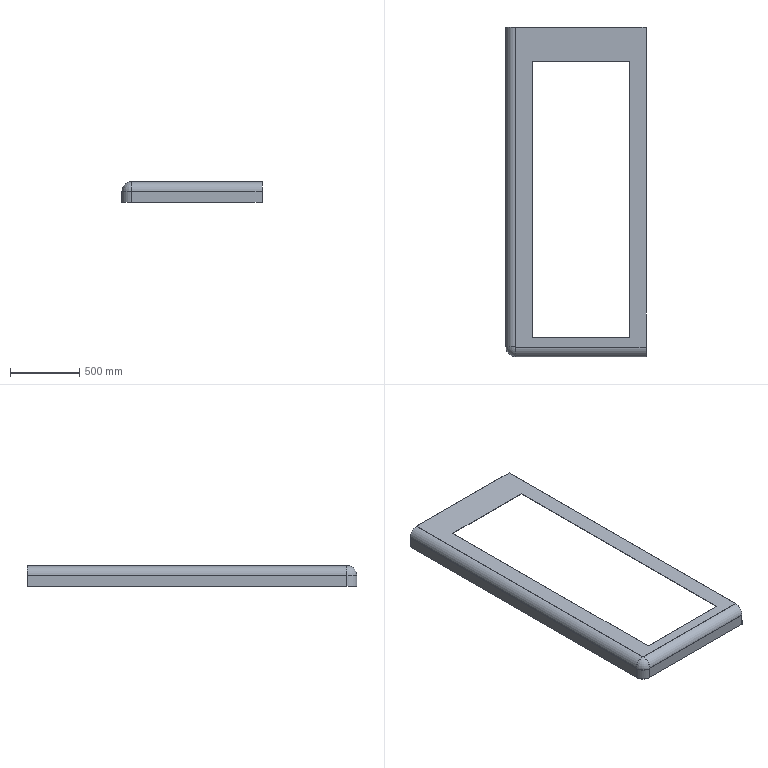Component | SolidWorks | A-SideAluminumCasingAssembly-1_A-SideAluminumCasing1-1 | 1 solid | 25 faces | box 1009.5 x 2375.5 x 149.5 mm | volume 4190304 mm3 | plane 17 | cylinder 6 | torus 2 | commonest cylinder face diameters 139 x2 133 x2 141 x1 135 x1
STEP:
#1=CARTESIAN_POINT('',(-0.2362,90.787,73.937));
#2=VERTEX_POINT('',#1);
#3=CARTESIAN_POINT('',(-0.2362,90.787,73.819));
#4=VERTEX_POINT('',#3);
#5=CARTESIAN_POINT('',(-0.2362,90.787,73.819));
#6=DIRECTION('',(0.,-0.,-1.));
#7=VECTOR('',#6,39.37);
#8=LINE('',#5,#7);
#9=EDGE_CURVE('',#2,#4,#8,.T.);
#10=ORIENTED_EDGE('',*,*,#9,.F.);
#11=CARTESIAN_POINT('',(-0.2362,0.,73.937));
#12=VERTEX_POINT('',#11);
#13=CARTESIAN_POINT('',(-0.2362,0.,73.937));
#14=DIRECTION('',(0.,-1.,0.));
#15=VECTOR('',#14,39.37);
#16=LINE('',#13,#15);
#17=EDGE_CURVE('',#2,#12,#16,.T.);
#18=ORIENTED_EDGE('',*,*,#17,.T.);
#19=CARTESIAN_POINT('',(-0.2362,0.,73.819));
#20=VERTEX_POINT('',#19);
#21=CARTESIAN_POINT('',(-0.2362,0.,73.819));
#22=DIRECTION('',(0.,-0.,-1.));
#23=VECTOR('',#22,39.37);
#24=LINE('',#21,#23);
#25=EDGE_CURVE('',#12,#20,#24,.T.);
#26=ORIENTED_EDGE('',*,*,#25,.T.);
#27=CARTESIAN_POINT('',(-0.2362,0.,73.819));
#28=DIRECTION('',(0.,-1.,0.));
#29=VECTOR('',#28,39.37);
#30=LINE('',#27,#29);
#31=EDGE_CURVE('',#4,#20,#30,.T.);
#32=ORIENTED_EDGE('',*,*,#31,.F.);
#33=EDGE_LOOP('',(#10,#18,#26,#32));
#34=FACE_OUTER_BOUND('',#33,.T.);
#35=CARTESIAN_POINT('',(-0.2362,0.,73.819));
#36=DIRECTION('',(1.,0.,0.));
#37=DIRECTION('',(0.,-1.,0.));
#38=AXIS2_PLACEMENT_3D('',#35,#36,#37);
#39=PLANE('',#38);
#40=ADVANCED_FACE('',(#34),#39,.T.);
#41=CARTESIAN_POINT('',(-37.244,90.787,73.937));
#42=VERTEX_POINT('',#41);
#43=CARTESIAN_POINT('',(-37.244,90.787,73.937));
#44=DIRECTION('',(1.,0.,0.));
#45=VECTOR('',#44,39.37);
#46=LINE('',#43,#45);
#47=EDGE_CURVE('',#42,#2,#46,.T.);
#48=ORIENTED_EDGE('',*,*,#47,.T.);
#49=ORIENTED_EDGE('',*,*,#9,.T.);
#50=CARTESIAN_POINT('',(-37.244,90.787,73.819));
#51=VERTEX_POINT('',#50);
#52=CARTESIAN_POINT('',(-37.244,90.787,73.819));
#53=DIRECTION('',(1.,0.,0.));
#54=VECTOR('',#53,39.37);
#55=LINE('',#52,#54);
#56=EDGE_CURVE('',#51,#4,#55,.T.);
#57=ORIENTED_EDGE('',*,*,#56,.F.);
#58=CARTESIAN_POINT('',(-37.244,90.787,73.819));
#59=DIRECTION('',(0.,-0.,-1.));
#60=VECTOR('',#59,39.37);
#61=LINE('',#58,#60);
#62=EDGE_CURVE('',#42,#51,#61,.T.);
#63=ORIENTED_EDGE('',*,*,#62,.F.);
#64=EDGE_LOOP('',(#48,#49,#57,#63));
#65=FACE_OUTER_BOUND('',#64,.T.);
#66=CARTESIAN_POINT('',(-37.244,90.787,73.819));
#67=DIRECTION('',(-0.,1.,-0.));
#68=DIRECTION('',(1.,0.,0.));
#69=AXIS2_PLACEMENT_3D('',#66,#67,#68);
#70=PLANE('',#69);
#71=ADVANCED_FACE('',(#65),#70,.T.);
#72=CARTESIAN_POINT('',(-32.48,2.736,73.819));
#73=VERTEX_POINT('',#72);
#74=CARTESIAN_POINT('',(-32.48,81.083,73.819));
#75=VERTEX_POINT('',#74);
#76=CARTESIAN_POINT('',(-32.48,0.,73.819));
#77=DIRECTION('',(-0.,1.,-0.));
#78=VECTOR('',#77,39.37);
#79=LINE('',#76,#78);
#80=EDGE_CURVE('',#73,#75,#79,.T.);
#81=ORIENTED_EDGE('',*,*,#80,.F.);
#82=CARTESIAN_POINT('',(-4.921,2.736,73.819));
#83=VERTEX_POINT('',#82);
#84=CARTESIAN_POINT('',(-37.244,2.736,73.819));
#85=DIRECTION('',(-1.,-0.,-0.));
#86=VECTOR('',#85,39.37);
#87=LINE('',#84,#86);
#88=EDGE_CURVE('',#83,#73,#87,.T.);
#89=ORIENTED_EDGE('',*,*,#88,.F.);
#90=CARTESIAN_POINT('',(-4.921,81.083,73.819));
#91=VERTEX_POINT('',#90);
#92=CARTESIAN_POINT('',(-4.921,0.,73.819));
#93=DIRECTION('',(0.,-1.,0.));
#94=VECTOR('',#93,39.37);
#95=LINE('',#92,#94);
#96=EDGE_CURVE('',#91,#83,#95,.T.);
#97=ORIENTED_EDGE('',*,*,#96,.F.);
#98=CARTESIAN_POINT('',(-37.244,81.083,73.819));
#99=DIRECTION('',(1.,0.,0.));
#100=VECTOR('',#99,39.37);
#101=LINE('',#98,#100);
#102=EDGE_CURVE('',#75,#91,#101,.T.);
#103=ORIENTED_EDGE('',*,*,#102,.F.);
#104=EDGE_LOOP('',(#81,#89,#97,#103));
#105=FACE_BOUND('',#104,.T.);
#106=CARTESIAN_POINT('',(-37.205,0.,73.819));
#107=VERTEX_POINT('',#106);
#108=CARTESIAN_POINT('',(-37.244,0.,73.819));
#109=DIRECTION('',(-1.,-0.,-0.));
#110=VECTOR('',#109,39.37);
#111=LINE('',#108,#110);
#112=EDGE_CURVE('',#20,#107,#111,.T.);
#113=ORIENTED_EDGE('',*,*,#112,.T.);
#114=CARTESIAN_POINT('',(-37.244,0.03937,73.819));
#115=VERTEX_POINT('',#114);
#116=CARTESIAN_POINT('',(-37.205,0.03937,73.819));
#117=DIRECTION('',(0.,-0.,-1.));
#118=DIRECTION('',(-1.,-0.,0.));
#119=AXIS2_PLACEMENT_3D('',#116,#117,#118);
#120=CIRCLE('',#119,0.03937);
#121=EDGE_CURVE('',#107,#115,#120,.T.);
#122=ORIENTED_EDGE('',*,*,#121,.T.);
#123=CARTESIAN_POINT('',(-37.244,0.,73.819));
#124=DIRECTION('',(-0.,1.,-0.));
#125=VECTOR('',#124,39.37);
#126=LINE('',#123,#125);
#127=EDGE_CURVE('',#115,#51,#126,.T.);
#128=ORIENTED_EDGE('',*,*,#127,.T.);
#129=ORIENTED_EDGE('',*,*,#56,.T.);
#130=ORIENTED_EDGE('',*,*,#31,.T.);
#131=EDGE_LOOP('',(#113,#122,#128,#129,#130));
#132=FACE_OUTER_BOUND('',#131,.T.);
#133=CARTESIAN_POINT('',(-37.244,0.,73.819));
#134=DIRECTION('',(0.,-0.,-1.));
#135=DIRECTION('',(-1.,-0.,-0.));
#136=AXIS2_PLACEMENT_3D('',#133,#134,#135);
#137=PLANE('',#136);
#138=ADVANCED_FACE('',(#105,#132),#137,.T.);
#139=CARTESIAN_POINT('',(-32.48,2.736,73.937));
#140=VERTEX_POINT('',#139);
#141=CARTESIAN_POINT('',(-4.921,2.736,73.937));
#142=VERTEX_POINT('',#141);
#143=CARTESIAN_POINT('',(-32.48,2.736,73.937));
#144=DIRECTION('',(1.,0.,0.));
#145=VECTOR('',#144,39.37);
#146=LINE('',#143,#145);
#147=EDGE_CURVE('',#140,#142,#146,.T.);
#148=ORIENTED_EDGE('',*,*,#147,.F.);
#149=CARTESIAN_POINT('',(-32.48,81.083,73.937));
#150=VERTEX_POINT('',#149);
#151=CARTESIAN_POINT('',(-32.48,2.736,73.937));
#152=DIRECTION('',(0.,-1.,0.));
#153=VECTOR('',#152,39.37);
#154=LINE('',#151,#153);
#155=EDGE_CURVE('',#150,#140,#154,.T.);
#156=ORIENTED_EDGE('',*,*,#155,.F.);
#157=CARTESIAN_POINT('',(-4.921,81.083,73.937));
#158=VERTEX_POINT('',#157);
#159=CARTESIAN_POINT('',(-32.48,81.083,73.937));
#160=DIRECTION('',(-1.,-0.,-0.));
#161=VECTOR('',#160,39.37);
#162=LINE('',#159,#161);
#163=EDGE_CURVE('',#158,#150,#162,.T.);
#164=ORIENTED_EDGE('',*,*,#163,.F.);
#165=CARTESIAN_POINT('',(-4.921,2.736,73.937));
#166=DIRECTION('',(-0.,1.,-0.));
#167=VECTOR('',#166,39.37);
#168=LINE('',#165,#167);
#169=EDGE_CURVE('',#142,#158,#168,.T.);
#170=ORIENTED_EDGE('',*,*,#169,.F.);
#171=EDGE_LOOP('',(#148,#156,#164,#170));
#172=FACE_BOUND('',#171,.T.);
#173=CARTESIAN_POINT('',(-37.244,0.03937,73.937));
#174=VERTEX_POINT('',#173);
#175=CARTESIAN_POINT('',(-37.244,0.,73.937));
#176=DIRECTION('',(-0.,1.,-0.));
#177=VECTOR('',#176,39.37);
#178=LINE('',#175,#177);
#179=EDGE_CURVE('',#174,#42,#178,.T.);
#180=ORIENTED_EDGE('',*,*,#179,.F.);
#181=CARTESIAN_POINT('',(-37.205,0.,73.937));
#182=VERTEX_POINT('',#181);
#183=CARTESIAN_POINT('',(-37.205,0.03937,73.937));
#184=DIRECTION('',(-0.,0.,1.));
#185=DIRECTION('',(-1.,-0.,0.));
#186=AXIS2_PLACEMENT_3D('',#183,#184,#185);
#187=CIRCLE('',#186,0.03937);
#188=EDGE_CURVE('',#174,#182,#187,.T.);
#189=ORIENTED_EDGE('',*,*,#188,.T.);
#190=CARTESIAN_POINT('',(-37.244,0.,73.937));
#191=DIRECTION('',(-1.,-0.,-0.));
#192=VECTOR('',#191,39.37);
#193=LINE('',#190,#192);
#194=EDGE_CURVE('',#12,#182,#193,.T.);
#195=ORIENTED_EDGE('',*,*,#194,.F.);
#196=ORIENTED_EDGE('',*,*,#17,.F.);
#197=ORIENTED_EDGE('',*,*,#47,.F.);
#198=EDGE_LOOP('',(#180,#189,#195,#196,#197));
#199=FACE_OUTER_BOUND('',#198,.T.);
#200=CARTESIAN_POINT('',(-37.244,0.,73.937));
#201=DIRECTION('',(0.,-0.,-1.));
#202=DIRECTION('',(-1.,-0.,-0.));
#203=AXIS2_PLACEMENT_3D('',#200,#201,#202);
#204=PLANE('',#203);
#205=ADVANCED_FACE('',(#172,#199),#204,.F.);
#206=CARTESIAN_POINT('',(-0.2362,-2.618,71.201));
#207=VERTEX_POINT('',#206);
#208=CARTESIAN_POINT('',(-0.2362,-2.736,71.201));
#209=VERTEX_POINT('',#208);
#210=CARTESIAN_POINT('',(-0.2362,-2.736,71.201));
#211=DIRECTION('',(0.,-1.,0.));
#212=VECTOR('',#211,39.37);
#213=LINE('',#210,#212);
#214=EDGE_CURVE('',#207,#209,#213,.T.);
#215=ORIENTED_EDGE('',*,*,#214,.F.);
#216=CARTESIAN_POINT('',(-0.2362,0.,71.201));
#217=DIRECTION('',(1.,0.,0.));
#218=DIRECTION('',(-0.,0.,1.));
#219=AXIS2_PLACEMENT_3D('',#216,#217,#218);
#220=CIRCLE('',#219,2.618);
#221=EDGE_CURVE('',#20,#207,#220,.T.);
#222=ORIENTED_EDGE('',*,*,#221,.F.);
#223=ORIENTED_EDGE('',*,*,#25,.F.);
#224=CARTESIAN_POINT('',(-0.2362,0.,71.201));
#225=DIRECTION('',(1.,0.,0.));
#226=DIRECTION('',(-0.,0.,1.));
#227=AXIS2_PLACEMENT_3D('',#224,#225,#226);
#228=CIRCLE('',#227,2.736);
#229=EDGE_CURVE('',#12,#209,#228,.T.);
#230=ORIENTED_EDGE('',*,*,#229,.T.);
#231=EDGE_LOOP('',(#215,#222,#223,#230));
#232=FACE_OUTER_BOUND('',#231,.T.);
#233=CARTESIAN_POINT('',(-0.2362,0.,71.201));
#234=DIRECTION('',(1.,0.,0.));
#235=DIRECTION('',(0.,-0.,-1.));
#236=AXIS2_PLACEMENT_3D('',#233,#234,#235);
#237=PLANE('',#236);
#238=ADVANCED_FACE('',(#232),#237,.T.);
#239=ORIENTED_EDGE('',*,*,#194,.T.);
#240=CARTESIAN_POINT('',(-37.205,-2.736,71.201));
#241=VERTEX_POINT('',#240);
#242=CARTESIAN_POINT('',(-37.205,0.,71.201));
#243=DIRECTION('',(-1.,-0.,-0.));
#244=DIRECTION('',(0.,0.,1.));
#245=AXIS2_PLACEMENT_3D('',#242,#243,#244);
#246=CIRCLE('',#245,2.736);
#247=EDGE_CURVE('',#241,#182,#246,.T.);
#248=ORIENTED_EDGE('',*,*,#247,.F.);
#249=CARTESIAN_POINT('',(-0.2362,-2.736,71.201));
#250=DIRECTION('',(1.,0.,0.));
#251=VECTOR('',#250,39.37);
#252=LINE('',#249,#251);
#253=EDGE_CURVE('',#241,#209,#252,.T.);
#254=ORIENTED_EDGE('',*,*,#253,.T.);
#255=ORIENTED_EDGE('',*,*,#229,.F.);
#256=EDGE_LOOP('',(#239,#248,#254,#255));
#257=FACE_OUTER_BOUND('',#256,.T.);
#258=CARTESIAN_POINT('',(-37.205,0.,71.201));
#259=DIRECTION('',(-1.,-0.,-0.));
#260=DIRECTION('',(0.,-1.,0.));
#261=AXIS2_PLACEMENT_3D('',#258,#259,#260);
#262=CYLINDRICAL_SURFACE('',#261,2.736);
#263=ADVANCED_FACE('',(#257),#262,.T.);
#264=ORIENTED_EDGE('',*,*,#112,.F.);
#265=ORIENTED_EDGE('',*,*,#221,.T.);
#266=CARTESIAN_POINT('',(-37.205,-2.618,71.201));
#267=VERTEX_POINT('',#266);
#268=CARTESIAN_POINT('',(-0.2362,-2.618,71.201));
#269=DIRECTION('',(-1.,-0.,-0.));
#270=VECTOR('',#269,39.37);
#271=LINE('',#268,#270);
#272=EDGE_CURVE('',#207,#267,#271,.T.);
#273=ORIENTED_EDGE('',*,*,#272,.T.);
#274=CARTESIAN_POINT('',(-37.205,0.,71.201));
#275=DIRECTION('',(-1.,-0.,-0.));
#276=DIRECTION('',(0.,0.,1.));
#277=AXIS2_PLACEMENT_3D('',#274,#275,#276);
#278=CIRCLE('',#277,2.618);
#279=EDGE_CURVE('',#267,#107,#278,.T.);
#280=ORIENTED_EDGE('',*,*,#279,.T.);
#281=EDGE_LOOP('',(#264,#265,#273,#280));
#282=FACE_OUTER_BOUND('',#281,.T.);
#283=CARTESIAN_POINT('',(-37.205,0.,71.201));
#284=DIRECTION('',(-1.,-0.,-0.));
#285=DIRECTION('',(0.,-1.,0.));
#286=AXIS2_PLACEMENT_3D('',#283,#284,#285);
#287=CYLINDRICAL_SURFACE('',#286,2.618);
#288=ADVANCED_FACE('',(#282),#287,.F.);
#289=ORIENTED_EDGE('',*,*,#214,.T.);
#290=CARTESIAN_POINT('',(-0.2362,-2.736,68.051));
#291=VERTEX_POINT('',#290);
#292=CARTESIAN_POINT('',(-0.2362,-2.736,73.819));
#293=DIRECTION('',(-0.,0.,1.));
#294=VECTOR('',#293,39.37);
#295=LINE('',#292,#294);
#296=EDGE_CURVE('',#291,#209,#295,.T.);
#297=ORIENTED_EDGE('',*,*,#296,.F.);
#298=CARTESIAN_POINT('',(-0.2362,-2.618,68.051));
#299=VERTEX_POINT('',#298);
#300=CARTESIAN_POINT('',(-0.2362,-2.736,68.051));
#301=DIRECTION('',(-0.,1.,-0.));
#302=VECTOR('',#301,39.37);
#303=LINE('',#300,#302);
#304=EDGE_CURVE('',#291,#299,#303,.T.);
#305=ORIENTED_EDGE('',*,*,#304,.T.);
#306=CARTESIAN_POINT('',(-0.2362,-2.618,73.819));
#307=DIRECTION('',(-0.,0.,1.));
#308=VECTOR('',#307,39.37);
#309=LINE('',#306,#308);
#310=EDGE_CURVE('',#299,#207,#309,.T.);
#311=ORIENTED_EDGE('',*,*,#310,.T.);
#312=EDGE_LOOP('',(#289,#297,#305,#311));
#313=FACE_OUTER_BOUND('',#312,.T.);
#314=CARTESIAN_POINT('',(-0.2362,-2.736,73.819));
#315=DIRECTION('',(-1.,-0.,-0.));
#316=DIRECTION('',(-0.,0.,1.));
#317=AXIS2_PLACEMENT_3D('',#314,#315,#316);
#318=PLANE('',#317);
#319=ADVANCED_FACE('',(#313),#318,.F.);
#320=ORIENTED_EDGE('',*,*,#253,.F.);
#321=CARTESIAN_POINT('',(-37.205,-2.736,68.051));
#322=VERTEX_POINT('',#321);
#323=CARTESIAN_POINT('',(-37.205,-2.736,73.819));
#324=DIRECTION('',(0.,-0.,-1.));
#325=VECTOR('',#324,39.37);
#326=LINE('',#323,#325);
#327=EDGE_CURVE('',#241,#322,#326,.T.);
#328=ORIENTED_EDGE('',*,*,#327,.T.);
#329=CARTESIAN_POINT('',(-37.244,-2.736,68.051));
#330=DIRECTION('',(1.,0.,0.));
#331=VECTOR('',#330,39.37);
#332=LINE('',#329,#331);
#333=EDGE_CURVE('',#322,#291,#332,.T.);
#334=ORIENTED_EDGE('',*,*,#333,.T.);
#335=ORIENTED_EDGE('',*,*,#296,.T.);
#336=EDGE_LOOP('',(#320,#328,#334,#335));
#337=FACE_OUTER_BOUND('',#336,.T.);
#338=CARTESIAN_POINT('',(-37.244,-2.736,73.819));
#339=DIRECTION('',(-0.,1.,-0.));
#340=DIRECTION('',(0.,-0.,-1.));
#341=AXIS2_PLACEMENT_3D('',#338,#339,#340);
#342=PLANE('',#341);
#343=ADVANCED_FACE('',(#337),#342,.F.);
#344=CARTESIAN_POINT('',(-37.205,-2.618,68.051));
#345=VERTEX_POINT('',#344);
#346=CARTESIAN_POINT('',(-37.205,-2.618,68.051));
#347=DIRECTION('',(0.,-0.,-1.));
#348=VECTOR('',#347,39.37);
#349=LINE('',#346,#348);
#350=EDGE_CURVE('',#267,#345,#349,.T.);
#351=ORIENTED_EDGE('',*,*,#350,.F.);
#352=ORIENTED_EDGE('',*,*,#272,.F.);
#353=ORIENTED_EDGE('',*,*,#310,.F.);
#354=CARTESIAN_POINT('',(-0.2362,-2.618,68.051));
#355=DIRECTION('',(1.,0.,0.));
#356=VECTOR('',#355,39.37);
#357=LINE('',#354,#356);
#358=EDGE_CURVE('',#345,#299,#357,.T.);
#359=ORIENTED_EDGE('',*,*,#358,.F.);
#360=EDGE_LOOP('',(#351,#352,#353,#359));
#361=FACE_OUTER_BOUND('',#360,.T.);
#362=CARTESIAN_POINT('',(-37.244,-2.618,73.819));
#363=DIRECTION('',(-0.,1.,-0.));
#364=DIRECTION('',(0.,-0.,-1.));
#365=AXIS2_PLACEMENT_3D('',#362,#363,#364);
#366=PLANE('',#365);
#367=ADVANCED_FACE('',(#361),#366,.T.);
#368=ORIENTED_EDGE('',*,*,#358,.T.);
#369=ORIENTED_EDGE('',*,*,#304,.F.);
#370=ORIENTED_EDGE('',*,*,#333,.F.);
#371=CARTESIAN_POINT('',(-39.98,0.03937,68.051));
#372=VERTEX_POINT('',#371);
#373=CARTESIAN_POINT('',(-37.205,0.03937,68.051));
#374=DIRECTION('',(0.,-0.,-1.));
#375=DIRECTION('',(0.,-1.,0.));
#376=AXIS2_PLACEMENT_3D('',#373,#374,#375);
#377=CIRCLE('',#376,2.776);
#378=EDGE_CURVE('',#322,#372,#377,.T.);
#379=ORIENTED_EDGE('',*,*,#378,.T.);
#380=CARTESIAN_POINT('',(-39.98,90.787,68.051));
#381=VERTEX_POINT('',#380);
#382=CARTESIAN_POINT('',(-39.98,0.,68.051));
#383=DIRECTION('',(0.,-1.,0.));
#384=VECTOR('',#383,39.37);
#385=LINE('',#382,#384);
#386=EDGE_CURVE('',#381,#372,#385,.T.);
#387=ORIENTED_EDGE('',*,*,#386,.F.);
#388=CARTESIAN_POINT('',(-39.862,90.787,68.051));
#389=VERTEX_POINT('',#388);
#390=CARTESIAN_POINT('',(-39.98,90.787,68.051));
#391=DIRECTION('',(1.,0.,-0.));
#392=VECTOR('',#391,39.37);
#393=LINE('',#390,#392);
#394=EDGE_CURVE('',#381,#389,#393,.T.);
#395=ORIENTED_EDGE('',*,*,#394,.T.);
#396=CARTESIAN_POINT('',(-39.862,0.03937,68.051));
#397=VERTEX_POINT('',#396);
#398=CARTESIAN_POINT('',(-39.862,0.03937,68.051));
#399=DIRECTION('',(0.,-1.,0.));
#400=VECTOR('',#399,39.37);
#401=LINE('',#398,#400);
#402=EDGE_CURVE('',#389,#397,#401,.T.);
#403=ORIENTED_EDGE('',*,*,#402,.T.);
#404=CARTESIAN_POINT('',(-37.205,0.03937,68.051));
#405=DIRECTION('',(0.,-0.,-1.));
#406=DIRECTION('',(0.,-1.,0.));
#407=AXIS2_PLACEMENT_3D('',#404,#405,#406);
#408=CIRCLE('',#407,2.657);
#409=EDGE_CURVE('',#345,#397,#408,.T.);
#410=ORIENTED_EDGE('',*,*,#409,.F.);
#411=EDGE_LOOP('',(#368,#369,#370,#379,#387,#395,#403,#410));
#412=FACE_OUTER_BOUND('',#411,.T.);
#413=CARTESIAN_POINT('',(-0.2362,-2.736,68.051));
#414=DIRECTION('',(-0.,0.,1.));
#415=DIRECTION('',(-0.,1.,-0.));
#416=AXIS2_PLACEMENT_3D('',#413,#414,#415);
#417=PLANE('',#416);
#418=ADVANCED_FACE('',(#412),#417,.F.);
#419=CARTESIAN_POINT('',(-39.862,90.787,71.201));
#420=VERTEX_POINT('',#419);
#421=CARTESIAN_POINT('',(-37.244,90.787,71.201));
#422=DIRECTION('',(-0.,1.,-0.));
#423=DIRECTION('',(0.,-0.,-1.));
#424=AXIS2_PLACEMENT_3D('',#421,#422,#423);
#425=CIRCLE('',#424,2.618);
#426=EDGE_CURVE('',#420,#51,#425,.T.);
#427=ORIENTED_EDGE('',*,*,#426,.F.);
#428=CARTESIAN_POINT('',(-39.98,90.787,71.201));
#429=VERTEX_POINT('',#428);
#430=CARTESIAN_POINT('',(-39.862,90.787,71.201));
#431=DIRECTION('',(-1.,-0.,0.));
#432=VECTOR('',#431,39.37);
#433=LINE('',#430,#432);
#434=EDGE_CURVE('',#420,#429,#433,.T.);
#435=ORIENTED_EDGE('',*,*,#434,.T.);
#436=CARTESIAN_POINT('',(-37.244,90.787,71.201));
#437=DIRECTION('',(-0.,1.,-0.));
#438=DIRECTION('',(0.,-0.,-1.));
#439=AXIS2_PLACEMENT_3D('',#436,#437,#438);
#440=CIRCLE('',#439,2.736);
#441=EDGE_CURVE('',#429,#42,#440,.T.);
#442=ORIENTED_EDGE('',*,*,#441,.T.);
#443=ORIENTED_EDGE('',*,*,#62,.T.);
#444=EDGE_LOOP('',(#427,#435,#442,#443));
#445=FACE_OUTER_BOUND('',#444,.T.);
#446=CARTESIAN_POINT('',(-37.244,90.787,71.201));
#447=DIRECTION('',(0.,-1.,0.));
#448=DIRECTION('',(-0.,0.,1.));
#449=AXIS2_PLACEMENT_3D('',#446,#447,#448);
#450=PLANE('',#449);
#451=ADVANCED_FACE('',(#445),#450,.F.);
#452=ORIENTED_EDGE('',*,*,#179,.T.);
#453=ORIENTED_EDGE('',*,*,#441,.F.);
#454=CARTESIAN_POINT('',(-39.98,0.03937,71.201));
#455=VERTEX_POINT('',#454);
#456=CARTESIAN_POINT('',(-39.98,0.03937,71.201));
#457=DIRECTION('',(0.,-1.,0.));
#458=VECTOR('',#457,39.37);
#459=LINE('',#456,#458);
#460=EDGE_CURVE('',#429,#455,#459,.T.);
#461=ORIENTED_EDGE('',*,*,#460,.T.);
#462=CARTESIAN_POINT('',(-37.244,0.03937,71.201));
#463=DIRECTION('',(0.,-1.,0.));
#464=DIRECTION('',(0.,-0.,-1.));
#465=AXIS2_PLACEMENT_3D('',#462,#463,#464);
#466=CIRCLE('',#465,2.736);
#467=EDGE_CURVE('',#174,#455,#466,.T.);
#468=ORIENTED_EDGE('',*,*,#467,.F.);
#469=EDGE_LOOP('',(#452,#453,#461,#468));
#470=FACE_OUTER_BOUND('',#469,.T.);
#471=CARTESIAN_POINT('',(-37.244,90.787,71.201));
#472=DIRECTION('',(-0.,1.,-0.));
#473=DIRECTION('',(-1.,-0.,0.));
#474=AXIS2_PLACEMENT_3D('',#471,#472,#473);
#475=CYLINDRICAL_SURFACE('',#474,2.736);
#476=ADVANCED_FACE('',(#470),#475,.T.);
#477=ORIENTED_EDGE('',*,*,#127,.F.);
#478=CARTESIAN_POINT('',(-39.862,0.03937,71.201));
#479=VERTEX_POINT('',#478);
#480=CARTESIAN_POINT('',(-37.244,0.03937,71.201));
#481=DIRECTION('',(0.,-1.,0.));
#482=DIRECTION('',(0.,-0.,-1.));
#483=AXIS2_PLACEMENT_3D('',#480,#481,#482);
#484=CIRCLE('',#483,2.618);
#485=EDGE_CURVE('',#115,#479,#484,.T.);
#486=ORIENTED_EDGE('',*,*,#485,.T.);
#487=CARTESIAN_POINT('',(-39.862,0.03937,71.201));
#488=DIRECTION('',(-0.,1.,-0.));
#489=VECTOR('',#488,39.37);
#490=LINE('',#487,#489);
#491=EDGE_CURVE('',#479,#420,#490,.T.);
#492=ORIENTED_EDGE('',*,*,#491,.T.);
#493=ORIENTED_EDGE('',*,*,#426,.T.);
#494=EDGE_LOOP('',(#477,#486,#492,#493));
#495=FACE_OUTER_BOUND('',#494,.T.);
#496=CARTESIAN_POINT('',(-37.244,90.787,71.201));
#497=DIRECTION('',(-0.,1.,-0.));
#498=DIRECTION('',(-1.,-0.,0.));
#499=AXIS2_PLACEMENT_3D('',#496,#497,#498);
#500=CYLINDRICAL_SURFACE('',#499,2.618);
#501=ADVANCED_FACE('',(#495),#500,.F.);
#502=ORIENTED_EDGE('',*,*,#434,.F.);
#503=CARTESIAN_POINT('',(-39.862,90.787,68.051));
#504=DIRECTION('',(-0.,-0.,-1.));
#505=VECTOR('',#504,39.37);
#506=LINE('',#503,#505);
#507=EDGE_CURVE('',#420,#389,#506,.T.);
#508=ORIENTED_EDGE('',*,*,#507,.T.);
#509=ORIENTED_EDGE('',*,*,#394,.F.);
#510=CARTESIAN_POINT('',(-39.98,90.787,73.819));
#511=DIRECTION('',(-0.,-0.,-1.));
#512=VECTOR('',#511,39.37);
#513=LINE('',#510,#512);
#514=EDGE_CURVE('',#429,#381,#513,.T.);
#515=ORIENTED_EDGE('',*,*,#514,.F.);
#516=EDGE_LOOP('',(#502,#508,#509,#515));
#517=FACE_OUTER_BOUND('',#516,.T.);
#518=CARTESIAN_POINT('',(-39.98,90.787,68.051));
#519=DIRECTION('',(0.,-1.,0.));
#520=DIRECTION('',(-1.,-0.,-0.));
#521=AXIS2_PLACEMENT_3D('',#518,#519,#520);
#522=PLANE('',#521);
#523=ADVANCED_FACE('',(#517),#522,.F.);
#524=ORIENTED_EDGE('',*,*,#460,.F.);
#525=ORIENTED_EDGE('',*,*,#514,.T.);
#526=ORIENTED_EDGE('',*,*,#386,.T.);
#527=CARTESIAN_POINT('',(-39.98,0.03937,73.819));
#528=DIRECTION('',(0.,0.,1.));
#529=VECTOR('',#528,39.37);
#530=LINE('',#527,#529);
#531=EDGE_CURVE('',#372,#455,#530,.T.);
#532=ORIENTED_EDGE('',*,*,#531,.T.);
#533=EDGE_LOOP('',(#524,#525,#526,#532));
#534=FACE_OUTER_BOUND('',#533,.T.);
#535=CARTESIAN_POINT('',(-39.98,0.,73.819));
#536=DIRECTION('',(1.,0.,-0.));
#537=DIRECTION('',(-0.,-0.,-1.));
#538=AXIS2_PLACEMENT_3D('',#535,#536,#537);
#539=PLANE('',#538);
#540=ADVANCED_FACE('',(#534),#539,.F.);
#541=ORIENTED_EDGE('',*,*,#507,.F.);
#542=ORIENTED_EDGE('',*,*,#491,.F.);
#543=CARTESIAN_POINT('',(-39.862,0.03937,73.819));
#544=DIRECTION('',(0.,0.,1.));
#545=VECTOR('',#544,39.37);
#546=LINE('',#543,#545);
#547=EDGE_CURVE('',#397,#479,#546,.T.);
#548=ORIENTED_EDGE('',*,*,#547,.F.);
#549=ORIENTED_EDGE('',*,*,#402,.F.);
#550=EDGE_LOOP('',(#541,#542,#548,#549));
#551=FACE_OUTER_BOUND('',#550,.T.);
#552=CARTESIAN_POINT('',(-39.862,0.,73.819));
#553=DIRECTION('',(1.,0.,-0.));
#554=DIRECTION('',(-0.,-0.,-1.));
#555=AXIS2_PLACEMENT_3D('',#552,#553,#554);
#556=PLANE('',#555);
#557=ADVANCED_FACE('',(#551),#556,.T.);
#558=ORIENTED_EDGE('',*,*,#121,.F.);
#559=ORIENTED_EDGE('',*,*,#279,.F.);
#560=CARTESIAN_POINT('',(-37.205,0.03937,71.201));
#561=DIRECTION('',(0.,-0.,-1.));
#562=DIRECTION('',(0.,-1.,0.));
#563=AXIS2_PLACEMENT_3D('',#560,#561,#562);
#564=CIRCLE('',#563,2.657);
#565=EDGE_CURVE('',#267,#479,#564,.T.);
#566=ORIENTED_EDGE('',*,*,#565,.T.);
#567=ORIENTED_EDGE('',*,*,#485,.F.);
#568=EDGE_LOOP('',(#558,#559,#566,#567));
#569=FACE_OUTER_BOUND('',#568,.T.);
#570=CARTESIAN_POINT('',(-37.205,0.03937,71.201));
#571=DIRECTION('',(0.,-0.,-1.));
#572=DIRECTION('',(-1.,-0.,-0.));
#573=AXIS2_PLACEMENT_3D('',#570,#571,#572);
#574=TOROIDAL_SURFACE('',#573,0.03937,2.618);
#575=ADVANCED_FACE('',(#569),#574,.F.);
#576=CARTESIAN_POINT('',(-37.205,0.03937,71.201));
#577=DIRECTION('',(0.,-0.,-1.));
#578=DIRECTION('',(0.,-1.,0.));
#579=AXIS2_PLACEMENT_3D('',#576,#577,#578);
#580=CIRCLE('',#579,2.776);
#581=EDGE_CURVE('',#241,#455,#580,.T.);
#582=ORIENTED_EDGE('',*,*,#581,.F.);
#583=ORIENTED_EDGE('',*,*,#247,.T.);
#584=ORIENTED_EDGE('',*,*,#188,.F.);
#585=ORIENTED_EDGE('',*,*,#467,.T.);
#586=EDGE_LOOP('',(#582,#583,#584,#585));
#587=FACE_OUTER_BOUND('',#586,.T.);
#588=CARTESIAN_POINT('',(-37.205,0.03937,71.201));
#589=DIRECTION('',(0.,-0.,-1.));
#590=DIRECTION('',(-1.,-0.,-0.));
#591=AXIS2_PLACEMENT_3D('',#588,#589,#590);
#592=TOROIDAL_SURFACE('',#591,0.03937,2.736);
#593=ADVANCED_FACE('',(#587),#592,.T.);
#594=ORIENTED_EDGE('',*,*,#378,.F.);
#595=ORIENTED_EDGE('',*,*,#327,.F.);
#596=ORIENTED_EDGE('',*,*,#581,.T.);
#597=ORIENTED_EDGE('',*,*,#531,.F.);
#598=EDGE_LOOP('',(#594,#595,#596,#597));
#599=FACE_OUTER_BOUND('',#598,.T.);
#600=CARTESIAN_POINT('',(-37.205,0.03937,71.201));
#601=DIRECTION('',(0.,-0.,-1.));
#602=DIRECTION('',(-1.,-0.,0.));
#603=AXIS2_PLACEMENT_3D('',#600,#601,#602);
#604=CYLINDRICAL_SURFACE('',#603,2.776);
#605=ADVANCED_FACE('',(#599),#604,.T.);
#606=ORIENTED_EDGE('',*,*,#565,.F.);
#607=ORIENTED_EDGE('',*,*,#350,.T.);
#608=ORIENTED_EDGE('',*,*,#409,.T.);
#609=ORIENTED_EDGE('',*,*,#547,.T.);
#610=EDGE_LOOP('',(#606,#607,#608,#609));
#611=FACE_OUTER_BOUND('',#610,.T.);
#612=CARTESIAN_POINT('',(-37.205,0.03937,71.201));
#613=DIRECTION('',(0.,-0.,-1.));
#614=DIRECTION('',(-1.,-0.,0.));
#615=AXIS2_PLACEMENT_3D('',#612,#613,#614);
#616=CYLINDRICAL_SURFACE('',#615,2.657);
#617=ADVANCED_FACE('',(#611),#616,.F.);
#618=ORIENTED_EDGE('',*,*,#80,.T.);
#619=CARTESIAN_POINT('',(-32.48,81.083,73.543));
#620=DIRECTION('',(-0.,0.,1.));
#621=VECTOR('',#620,39.37);
#622=LINE('',#619,#621);
#623=EDGE_CURVE('',#75,#150,#622,.T.);
#624=ORIENTED_EDGE('',*,*,#623,.T.);
#625=ORIENTED_EDGE('',*,*,#155,.T.);
#626=CARTESIAN_POINT('',(-32.48,2.736,73.543));
#627=DIRECTION('',(-0.,0.,1.));
#628=VECTOR('',#627,39.37);
#629=LINE('',#626,#628);
#630=EDGE_CURVE('',#73,#140,#629,.T.);
#631=ORIENTED_EDGE('',*,*,#630,.F.);
#632=EDGE_LOOP('',(#618,#624,#625,#631));
#633=FACE_OUTER_BOUND('',#632,.T.);
#634=CARTESIAN_POINT('',(-32.48,2.736,73.543));
#635=DIRECTION('',(-1.,-0.,-0.));
#636=DIRECTION('',(-0.,0.,1.));
#637=AXIS2_PLACEMENT_3D('',#634,#635,#636);
#638=PLANE('',#637);
#639=ADVANCED_FACE('',(#633),#638,.F.);
#640=ORIENTED_EDGE('',*,*,#102,.T.);
#641=CARTESIAN_POINT('',(-4.921,81.083,73.543));
#642=DIRECTION('',(-0.,0.,1.));
#643=VECTOR('',#642,39.37);
#644=LINE('',#641,#643);
#645=EDGE_CURVE('',#91,#158,#644,.T.);
#646=ORIENTED_EDGE('',*,*,#645,.T.);
#647=ORIENTED_EDGE('',*,*,#163,.T.);
#648=ORIENTED_EDGE('',*,*,#623,.F.);
#649=EDGE_LOOP('',(#640,#646,#647,#648));
#650=FACE_OUTER_BOUND('',#649,.T.);
#651=CARTESIAN_POINT('',(-32.48,81.083,73.543));
#652=DIRECTION('',(-0.,1.,-0.));
#653=DIRECTION('',(0.,-0.,-1.));
#654=AXIS2_PLACEMENT_3D('',#651,#652,#653);
#655=PLANE('',#654);
#656=ADVANCED_FACE('',(#650),#655,.F.);
#657=ORIENTED_EDGE('',*,*,#96,.T.);
#658=CARTESIAN_POINT('',(-4.921,2.736,73.543));
#659=DIRECTION('',(-0.,0.,1.));
#660=VECTOR('',#659,39.37);
#661=LINE('',#658,#660);
#662=EDGE_CURVE('',#83,#142,#661,.T.);
#663=ORIENTED_EDGE('',*,*,#662,.T.);
#664=ORIENTED_EDGE('',*,*,#169,.T.);
#665=ORIENTED_EDGE('',*,*,#645,.F.);
#666=EDGE_LOOP('',(#657,#663,#664,#665));
#667=FACE_OUTER_BOUND('',#666,.T.);
#668=CARTESIAN_POINT('',(-4.921,2.736,73.543));
#669=DIRECTION('',(1.,0.,0.));
#670=DIRECTION('',(0.,-0.,-1.));
#671=AXIS2_PLACEMENT_3D('',#668,#669,#670);
#672=PLANE('',#671);
#673=ADVANCED_FACE('',(#667),#672,.F.);
#674=ORIENTED_EDGE('',*,*,#88,.T.);
#675=ORIENTED_EDGE('',*,*,#630,.T.);
#676=ORIENTED_EDGE('',*,*,#147,.T.);
#677=ORIENTED_EDGE('',*,*,#662,.F.);
#678=EDGE_LOOP('',(#674,#675,#676,#677));
#679=FACE_OUTER_BOUND('',#678,.T.);
#680=CARTESIAN_POINT('',(-32.48,2.736,73.543));
#681=DIRECTION('',(0.,-1.,0.));
#682=DIRECTION('',(-0.,0.,1.));
#683=AXIS2_PLACEMENT_3D('',#680,#681,#682);
#684=PLANE('',#683);
#685=ADVANCED_FACE('',(#679),#684,.F.);
#686=CLOSED_SHELL('',(#40,#71,#138,#205,#238,#263,#288,#319,#343,#367,#418,#451,#476,#501,#523,#540,#557,#575,#593,#605,#617,#639,#656,#673,#685));
#687=MANIFOLD_SOLID_BREP('',#686);
#688=CARTESIAN_POINT('',(0.,0.,0.));
#689=DIRECTION('',(0.,0.,1.));
#690=DIRECTION('',(1.,0.,0.));
#691=AXIS2_PLACEMENT_3D('',#688,#689,#690);
#692=(LENGTH_UNIT()NAMED_UNIT(*)SI_UNIT($,.METRE.));
#693=LENGTH_MEASURE_WITH_UNIT(LENGTH_MEASURE(0.0254),#692);
#694=DIMENSIONAL_EXPONENTS(1.,0.,0.,0.,0.,0.,0.);
#695=(CONVERSION_BASED_UNIT('',#693)LENGTH_UNIT()NAMED_UNIT(#694));
#696=UNCERTAINTY_MEASURE_WITH_UNIT(LENGTH_MEASURE(0.00001),#695,'','');
#697=(NAMED_UNIT(*)PLANE_ANGLE_UNIT()SI_UNIT($,.RADIAN.));
#698=(NAMED_UNIT(*)SI_UNIT($,.STERADIAN.)SOLID_ANGLE_UNIT());
#699=(GEOMETRIC_REPRESENTATION_CONTEXT(3)GLOBAL_UNCERTAINTY_ASSIGNED_CONTEXT((#696))GLOBAL_UNIT_ASSIGNED_CONTEXT((#695,#697,#698))REPRESENTATION_CONTEXT('',''));
#700=ADVANCED_BREP_SHAPE_REPRESENTATION('',(#687,#691),#699);
#701=COLOUR_RGB('',0.7922,0.8196,0.9333);
#702=FILL_AREA_STYLE_COLOUR('',#701);
#703=FILL_AREA_STYLE('',(#702));
#704=SURFACE_STYLE_FILL_AREA(#703);
#705=SURFACE_SIDE_STYLE('',(#704));
#706=SURFACE_STYLE_USAGE(.BOTH.,#705);
#707=PRESENTATION_STYLE_ASSIGNMENT((#706));
#708=STYLED_ITEM('',(#707),#687);
#709=(LENGTH_UNIT()NAMED_UNIT(*)SI_UNIT($,.METRE.));
#710=LENGTH_MEASURE_WITH_UNIT(LENGTH_MEASURE(0.0254),#709);
#711=DIMENSIONAL_EXPONENTS(1.,0.,0.,0.,0.,0.,0.);
#712=(CONVERSION_BASED_UNIT('',#710)LENGTH_UNIT()NAMED_UNIT(#711));
#713=UNCERTAINTY_MEASURE_WITH_UNIT(LENGTH_MEASURE(0.00001),#712,'','');
#714=(NAMED_UNIT(*)PLANE_ANGLE_UNIT()SI_UNIT($,.RADIAN.));
#715=(NAMED_UNIT(*)SI_UNIT($,.STERADIAN.)SOLID_ANGLE_UNIT());
#716=(GEOMETRIC_REPRESENTATION_CONTEXT(3)GLOBAL_UNCERTAINTY_ASSIGNED_CONTEXT((#713))GLOBAL_UNIT_ASSIGNED_CONTEXT((#712,#714,#715))REPRESENTATION_CONTEXT('',''));
#717=MECHANICAL_DESIGN_GEOMETRIC_PRESENTATION_REPRESENTATION('',(#708),#716);
#718=PRESENTATION_LAYER_ASSIGNMENT('','',(#708));